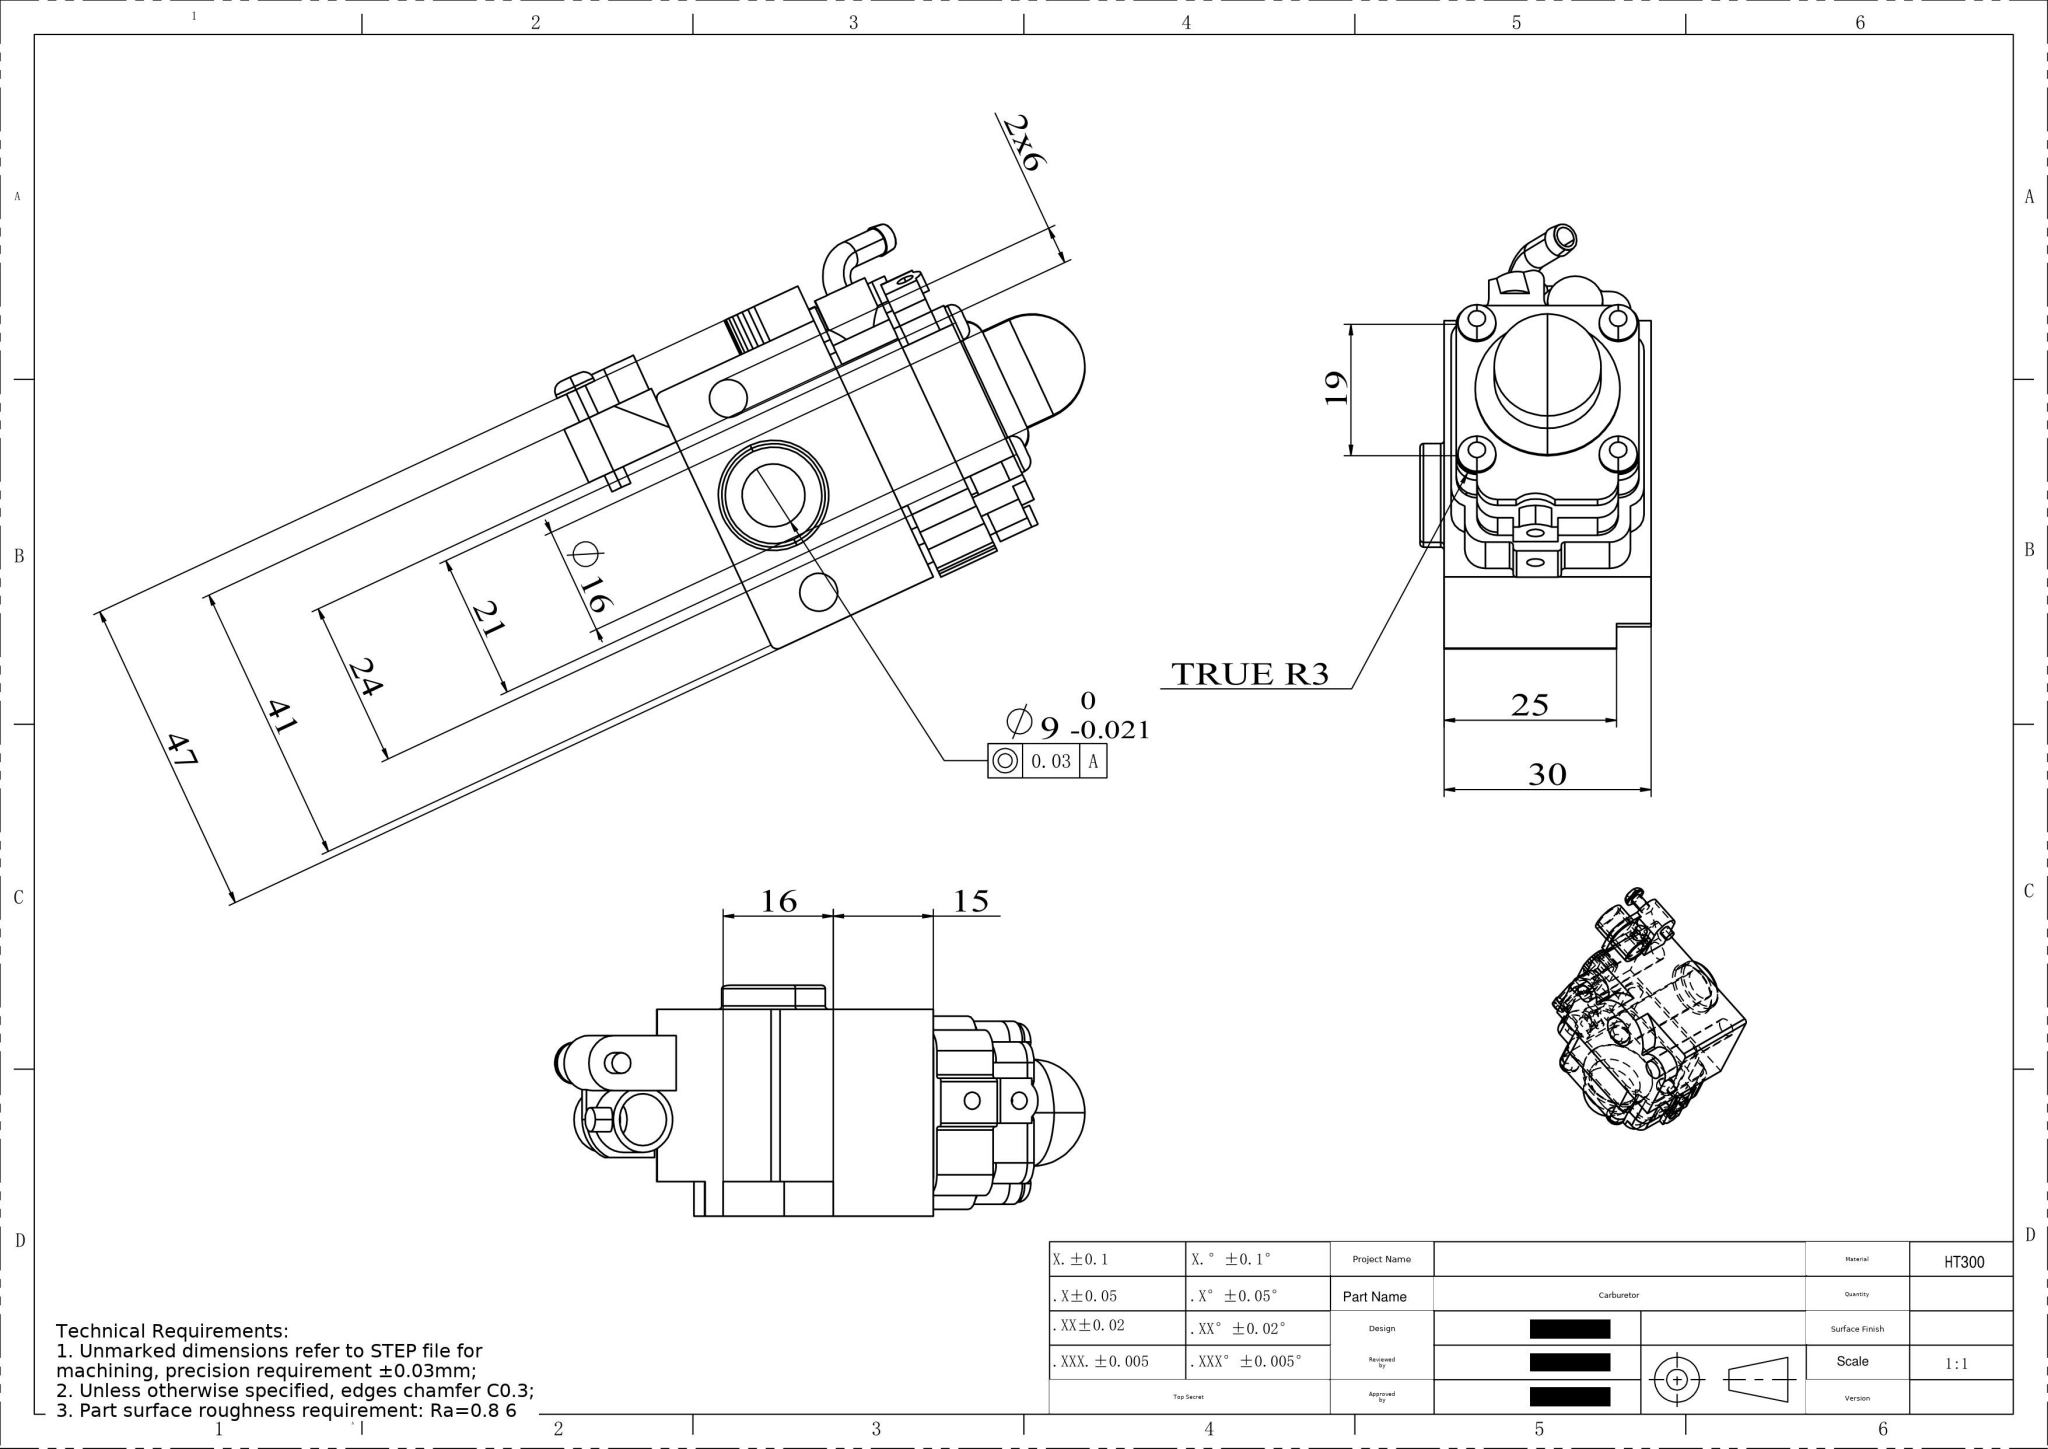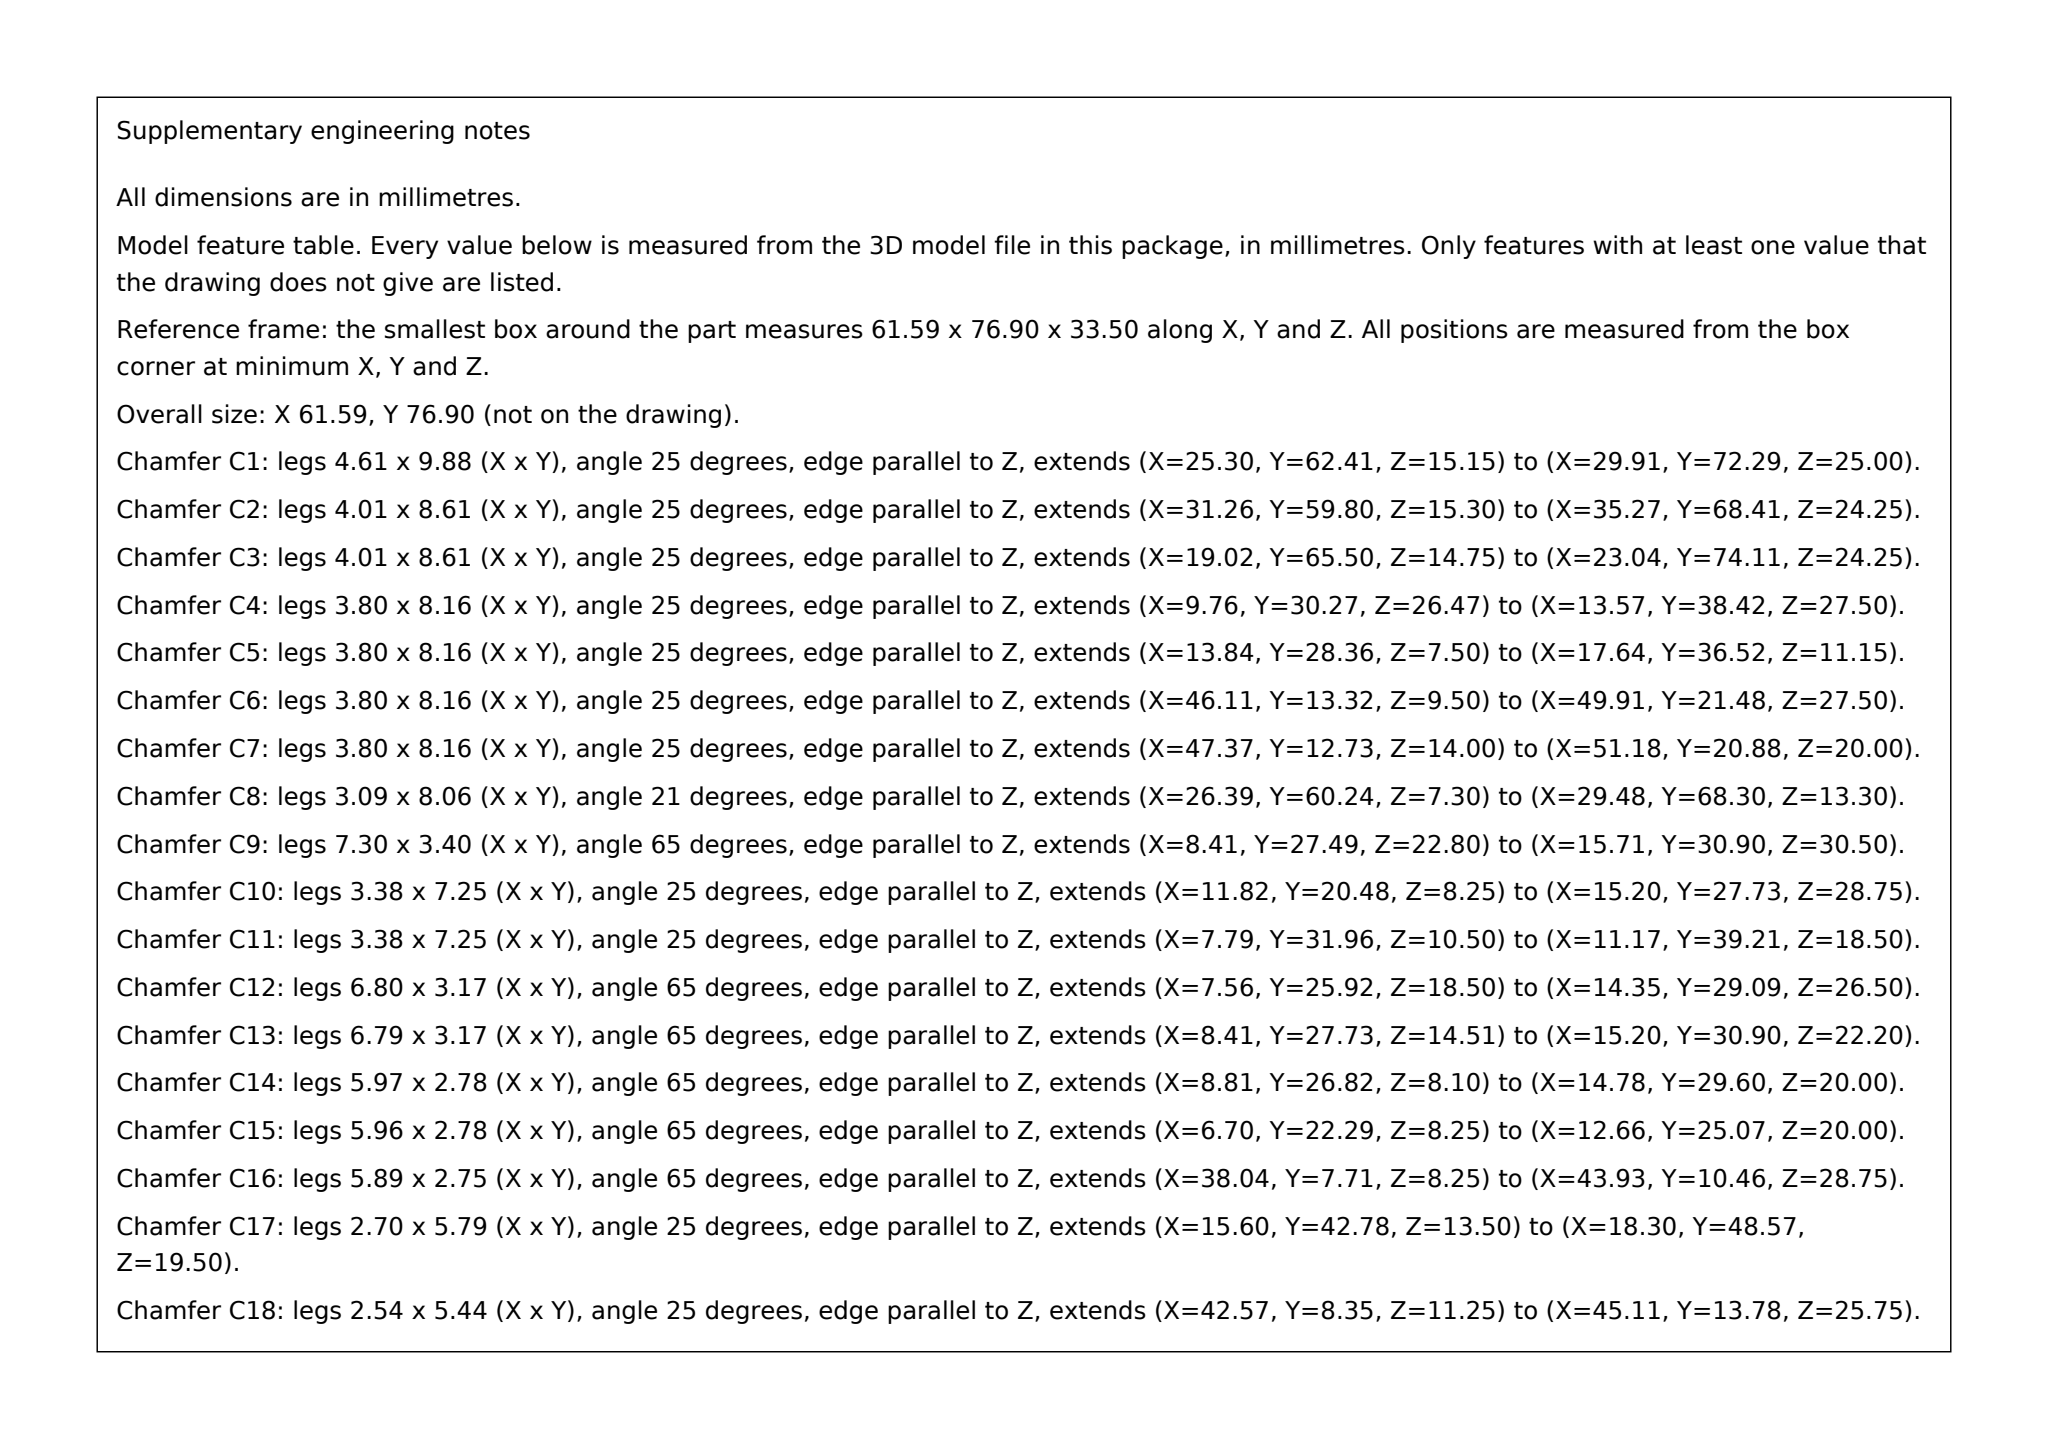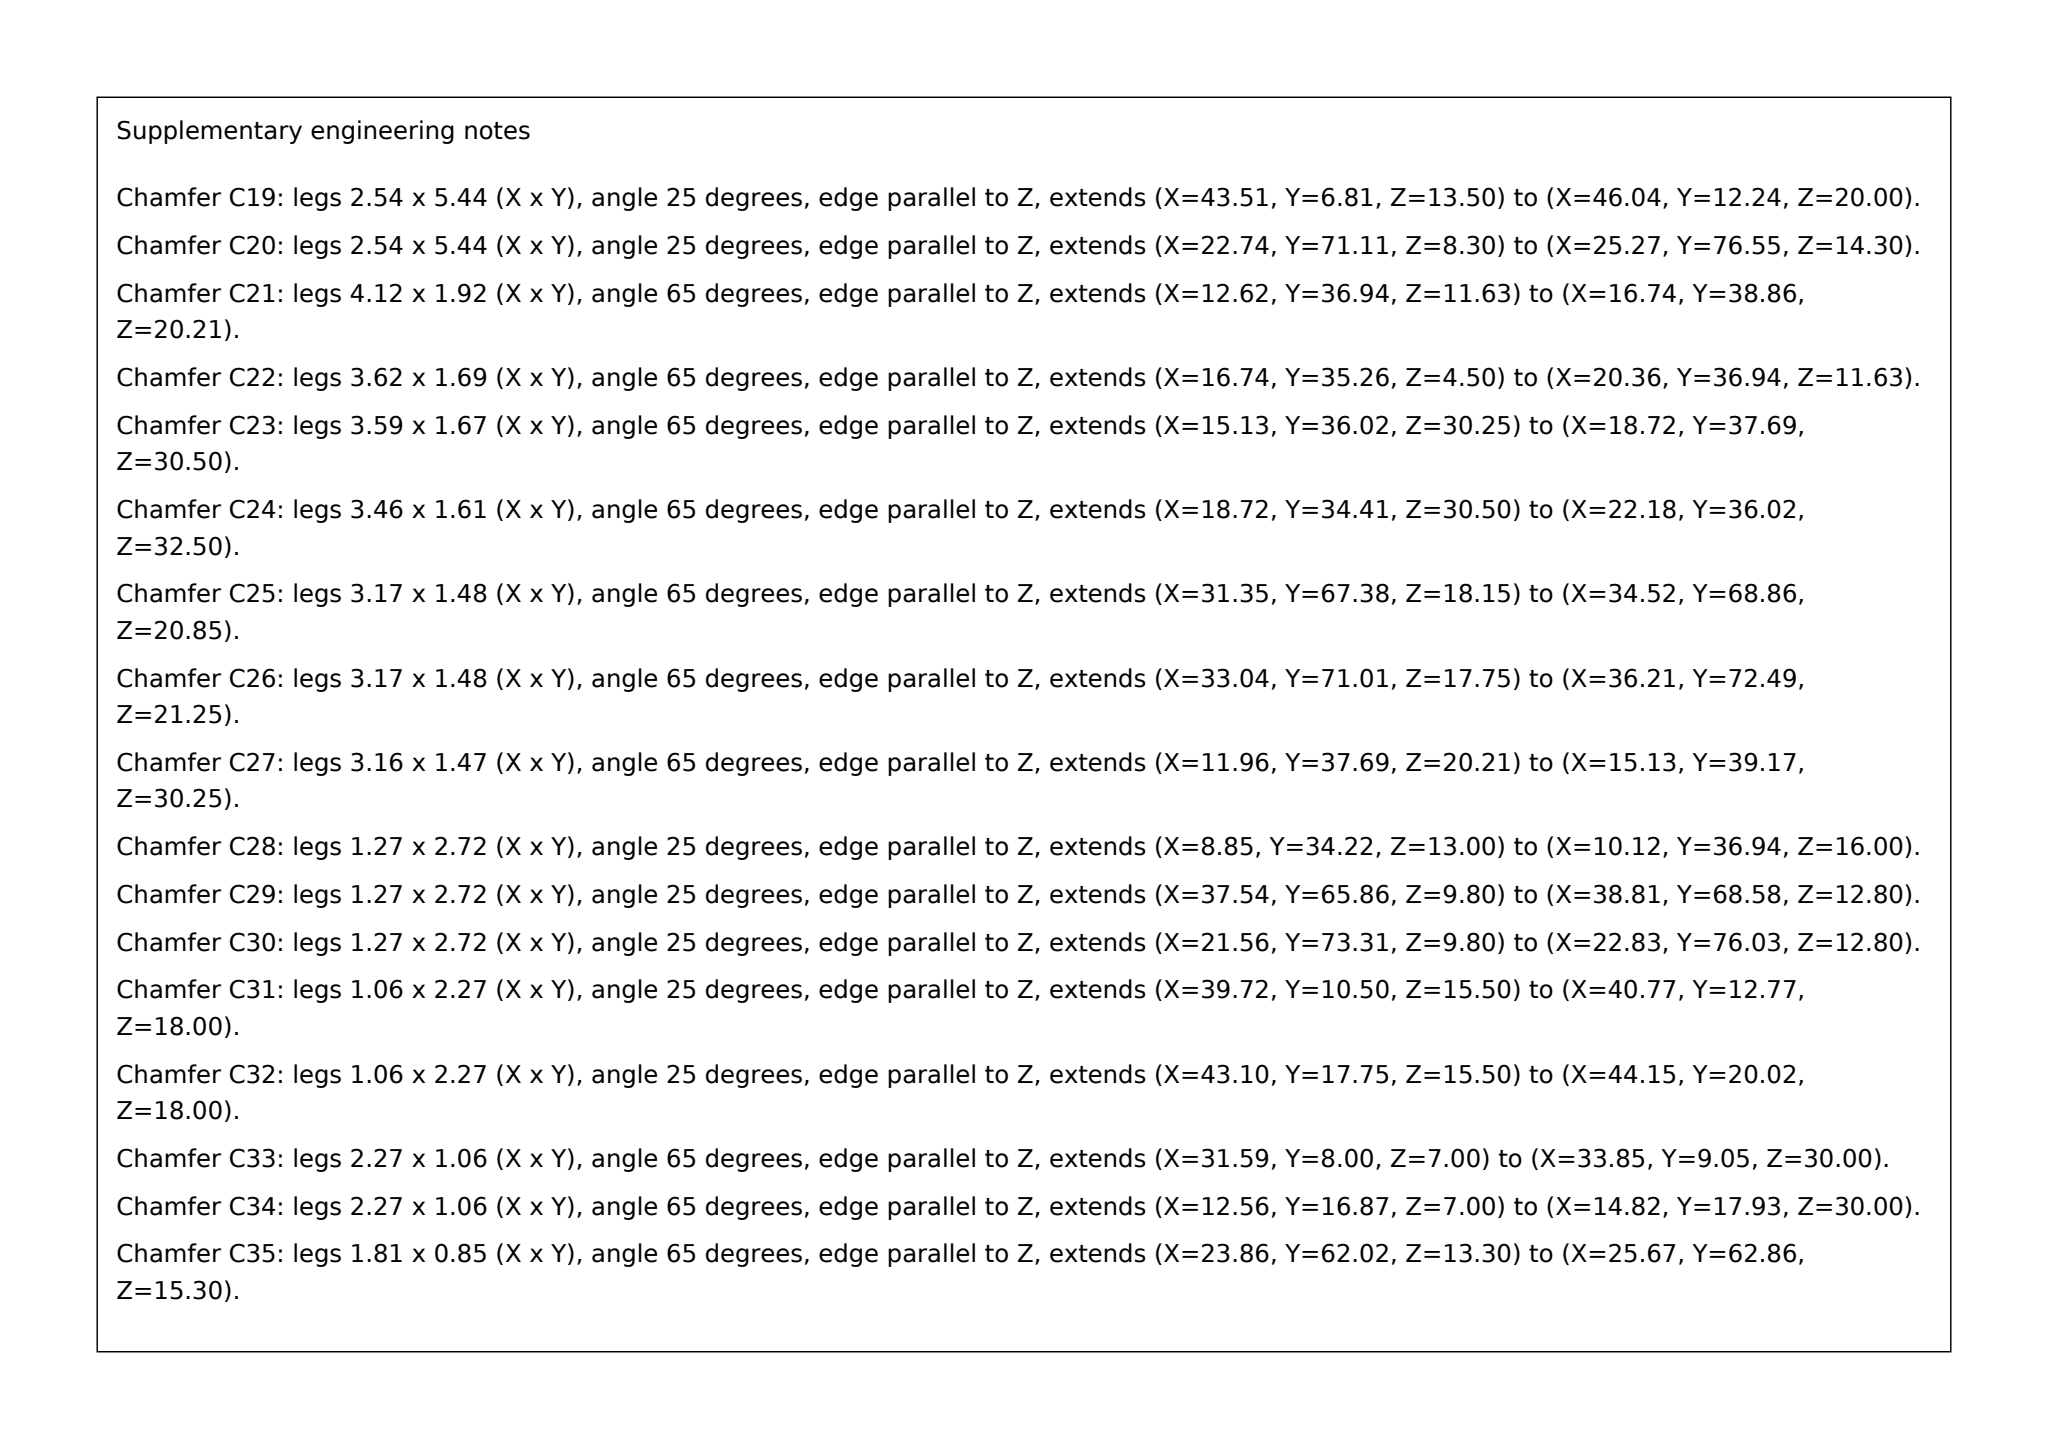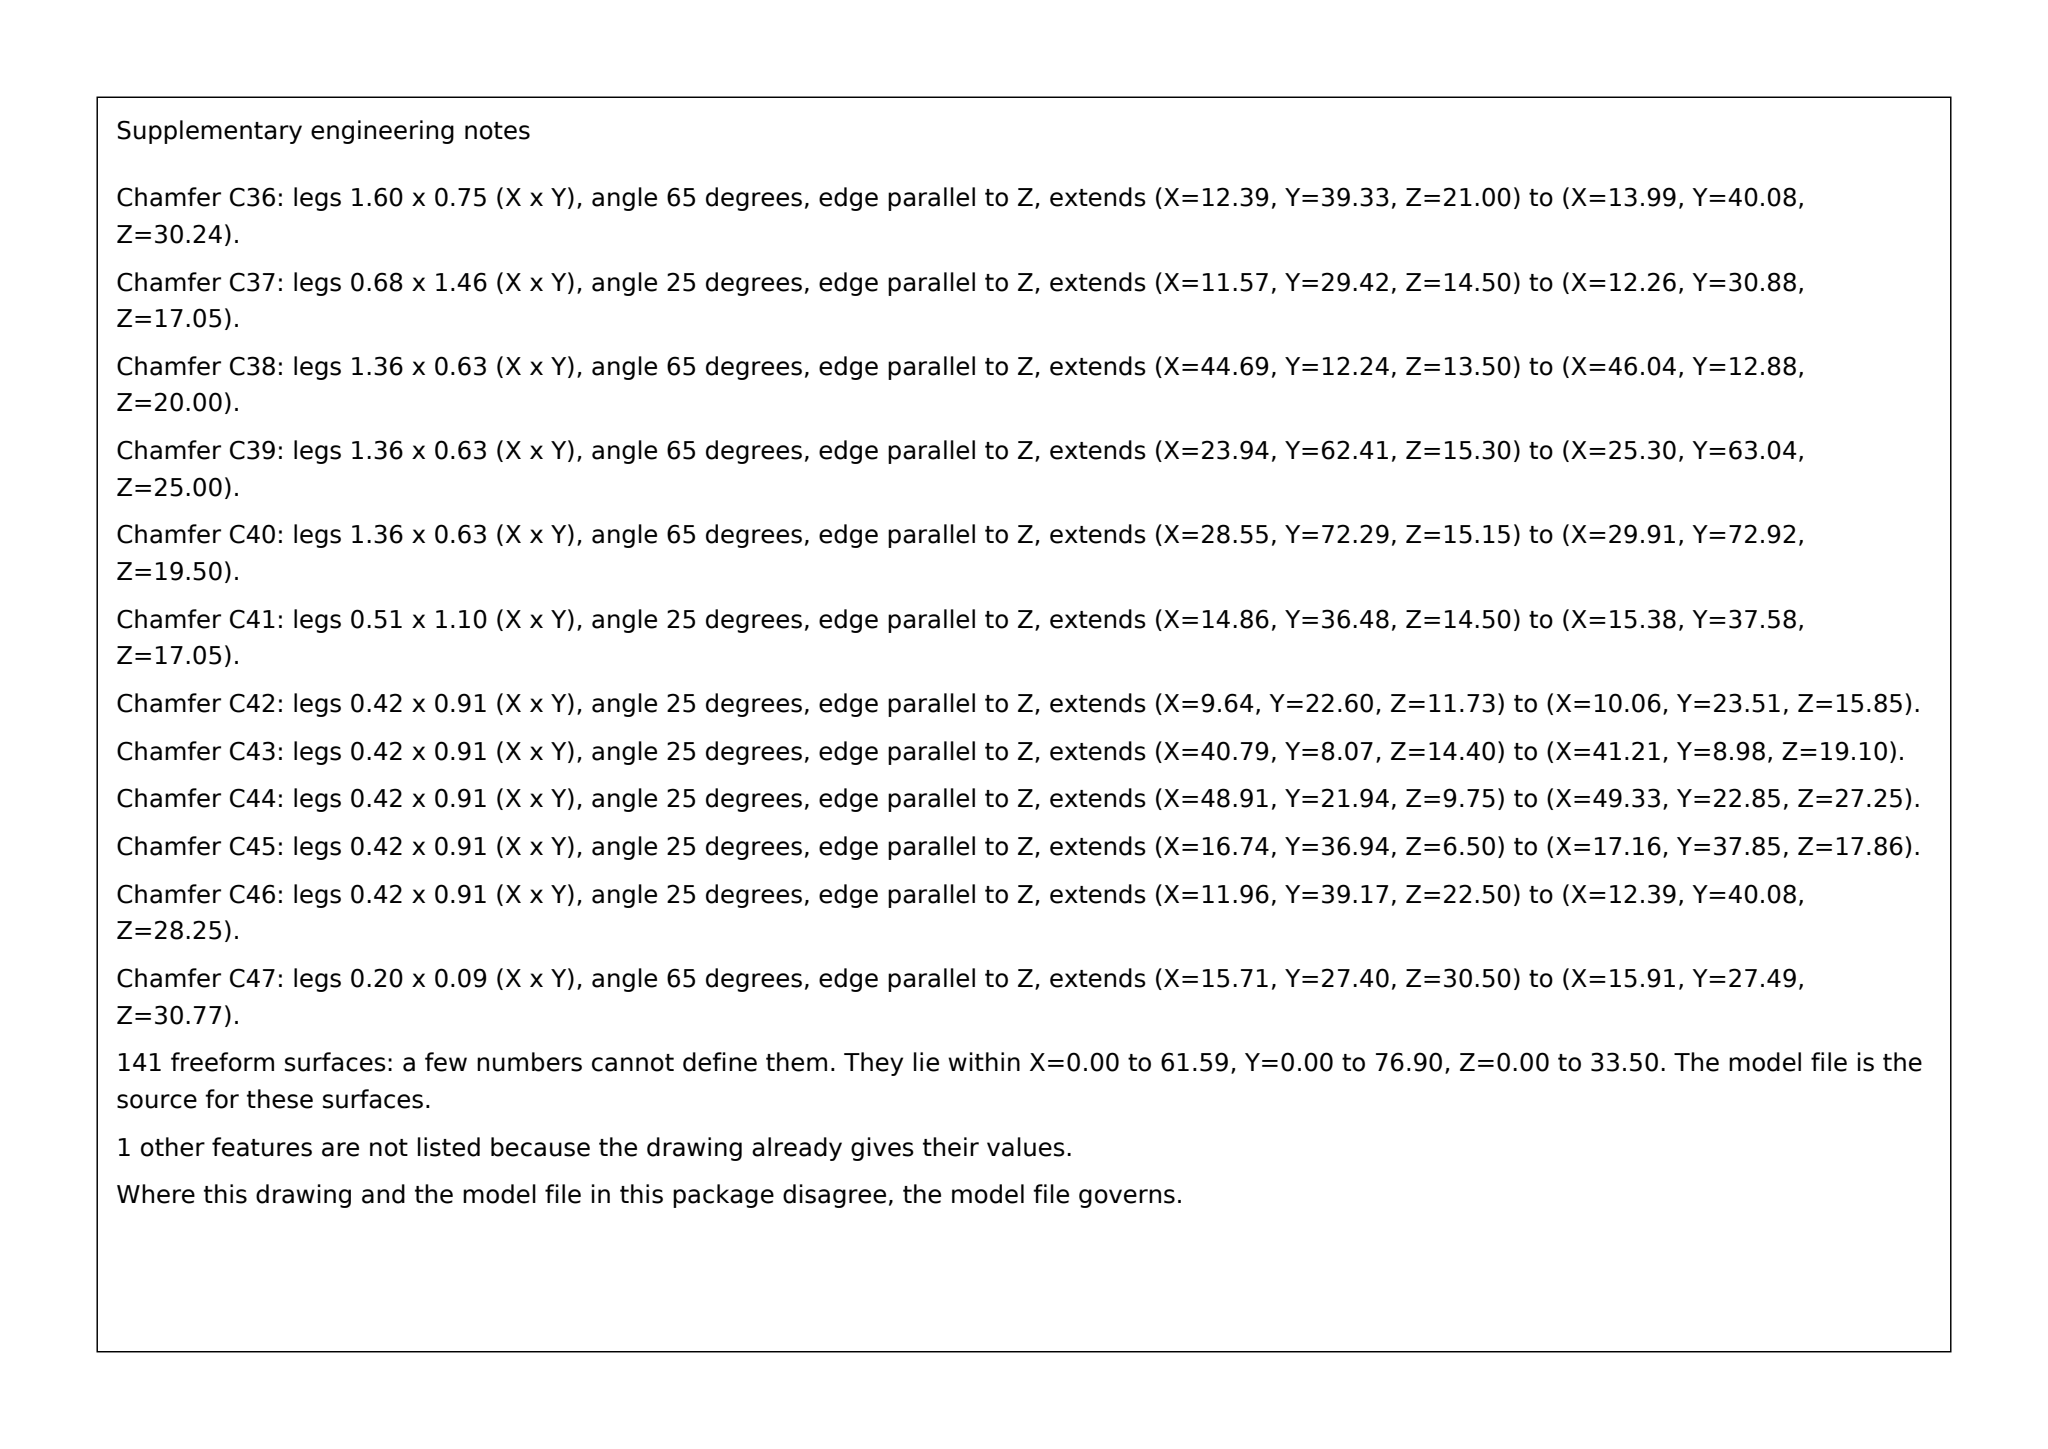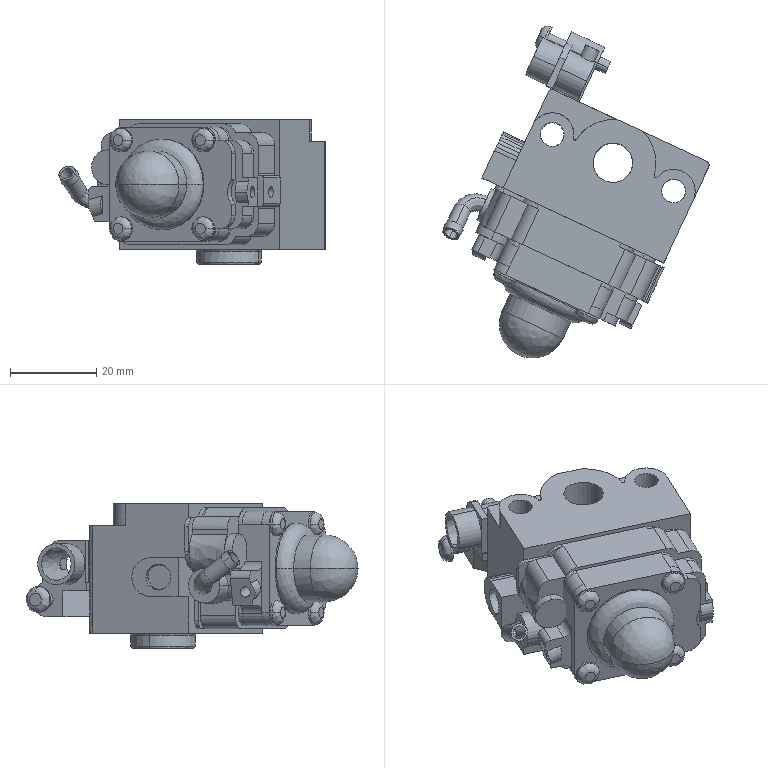Part | SolidWorks | mm | material HT300 | 1 solid | 254 faces | box 61.59 x 76.9 x 33.5 mm | volume 49916 mm3 | spline 141 | plane 113